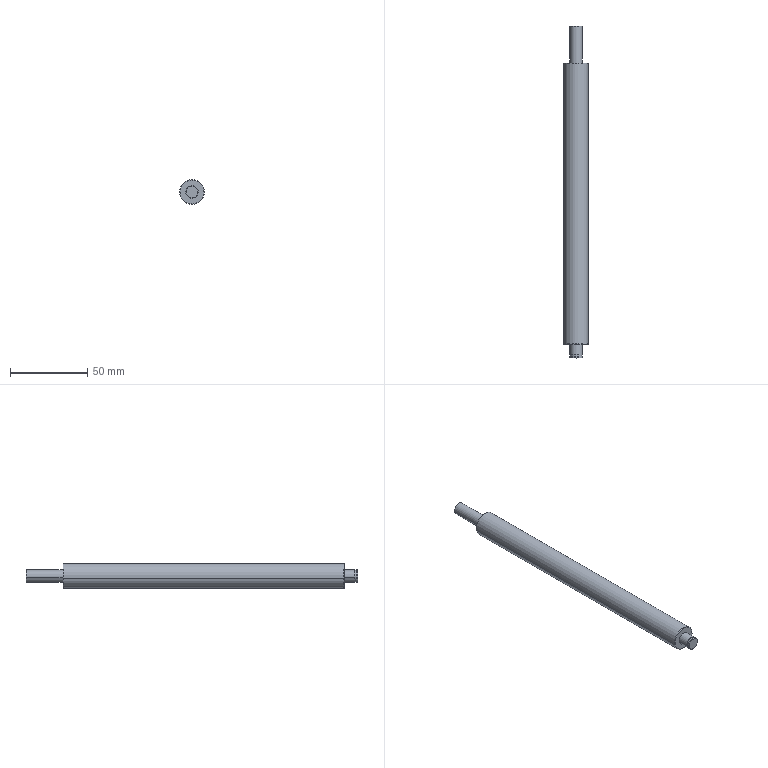Component | SolidWorks | 100-1_Copy(3)-1 | 1 solid | 24 faces | box 16 x 215 x 16 mm | volume 38242 mm3 | cylinder 10 | cone 8 | plane 6 | commonest cylinder face diameters 8 x6 7.4 x2 16 x2
STEP:
#1=COLOUR_RGB('',0.7922,0.8196,0.9333);
#2=FILL_AREA_STYLE_COLOUR('',#1);
#3=FILL_AREA_STYLE('',(#2));
#4=SURFACE_STYLE_FILL_AREA(#3);
#5=SURFACE_SIDE_STYLE('',(#4));
#6=SURFACE_STYLE_USAGE(.BOTH.,#5);
#7=PRESENTATION_STYLE_ASSIGNMENT((#6));
#8=CARTESIAN_POINT('',(19.273,49.724,-79.116));
#9=VERTEX_POINT('',#8);
#10=CARTESIAN_POINT('',(19.265,49.717,-79.117));
#11=VERTEX_POINT('',#10);
#12=CARTESIAN_POINT('',(19.273,49.724,-79.116));
#13=DIRECTION('',(-0.6974,-0.7071,-0.1169));
#14=VECTOR('',#13,39.37);
#15=LINE('',#12,#14);
#16=EDGE_CURVE('',#9,#11,#15,.T.);
#17=ORIENTED_EDGE('',*,*,#16,.F.);
#18=CARTESIAN_POINT('',(19.879,49.724,-79.014));
#19=VERTEX_POINT('',#18);
#20=CARTESIAN_POINT('',(19.576,49.724,-79.065));
#21=DIRECTION('',(-0.,1.,0.));
#22=DIRECTION('',(-0.9862,0.,-0.1654));
#23=AXIS2_PLACEMENT_3D('',#20,#21,#22);
#24=CIRCLE('',#23,0.3071);
#25=EDGE_CURVE('',#19,#9,#24,.T.);
#26=ORIENTED_EDGE('',*,*,#25,.F.);
#27=CARTESIAN_POINT('',(19.887,49.717,-79.013));
#28=VERTEX_POINT('',#27);
#29=CARTESIAN_POINT('',(19.879,49.724,-79.014));
#30=DIRECTION('',(0.6974,-0.7071,0.1169));
#31=VECTOR('',#30,39.37);
#32=LINE('',#29,#31);
#33=EDGE_CURVE('',#19,#28,#32,.T.);
#34=ORIENTED_EDGE('',*,*,#33,.T.);
#35=CARTESIAN_POINT('',(19.576,49.717,-79.065));
#36=DIRECTION('',(0.,-1.,-0.));
#37=DIRECTION('',(-0.9862,0.,-0.1654));
#38=AXIS2_PLACEMENT_3D('',#35,#36,#37);
#39=CIRCLE('',#38,0.315);
#40=EDGE_CURVE('',#11,#28,#39,.T.);
#41=ORIENTED_EDGE('',*,*,#40,.F.);
#42=EDGE_LOOP('',(#17,#26,#34,#41));
#43=FACE_OUTER_BOUND('',#42,.T.);
#44=CARTESIAN_POINT('',(19.576,49.724,-79.065));
#45=DIRECTION('',(0.,-1.,-0.));
#46=DIRECTION('',(0.9862,0.,0.1654));
#47=AXIS2_PLACEMENT_3D('',#44,#45,#46);
#48=CONICAL_SURFACE('',#47,0.3071,0.7854);
#49=ADVANCED_FACE('',(#43),#48,.T.);
#50=CARTESIAN_POINT('',(19.429,50.669,-79.09));
#51=VERTEX_POINT('',#50);
#52=CARTESIAN_POINT('',(19.421,50.661,-79.091));
#53=VERTEX_POINT('',#52);
#54=CARTESIAN_POINT('',(19.421,50.661,-79.091));
#55=DIRECTION('',(-0.6974,-0.7071,-0.1169));
#56=VECTOR('',#55,39.37);
#57=LINE('',#54,#56);
#58=EDGE_CURVE('',#51,#53,#57,.T.);
#59=ORIENTED_EDGE('',*,*,#58,.F.);
#60=CARTESIAN_POINT('',(19.724,50.669,-79.04));
#61=VERTEX_POINT('',#60);
#62=CARTESIAN_POINT('',(19.576,50.669,-79.065));
#63=DIRECTION('',(-0.,1.,0.));
#64=DIRECTION('',(-0.9862,0.,-0.1654));
#65=AXIS2_PLACEMENT_3D('',#62,#63,#64);
#66=CIRCLE('',#65,0.1496);
#67=EDGE_CURVE('',#61,#51,#66,.T.);
#68=ORIENTED_EDGE('',*,*,#67,.F.);
#69=CARTESIAN_POINT('',(19.731,50.661,-79.039));
#70=VERTEX_POINT('',#69);
#71=CARTESIAN_POINT('',(19.731,50.661,-79.039));
#72=DIRECTION('',(0.6974,-0.7071,0.1169));
#73=VECTOR('',#72,39.37);
#74=LINE('',#71,#73);
#75=EDGE_CURVE('',#61,#70,#74,.T.);
#76=ORIENTED_EDGE('',*,*,#75,.T.);
#77=CARTESIAN_POINT('',(19.576,50.661,-79.065));
#78=DIRECTION('',(0.,-1.,-0.));
#79=DIRECTION('',(-0.9862,0.,-0.1654));
#80=AXIS2_PLACEMENT_3D('',#77,#78,#79);
#81=CIRCLE('',#80,0.1575);
#82=EDGE_CURVE('',#53,#70,#81,.T.);
#83=ORIENTED_EDGE('',*,*,#82,.F.);
#84=EDGE_LOOP('',(#59,#68,#76,#83));
#85=FACE_OUTER_BOUND('',#84,.T.);
#86=CARTESIAN_POINT('',(19.576,50.661,-79.065));
#87=DIRECTION('',(0.,-1.,-0.));
#88=DIRECTION('',(0.9862,0.,0.1654));
#89=AXIS2_PLACEMENT_3D('',#86,#87,#88);
#90=CONICAL_SURFACE('',#89,0.1575,0.7854);
#91=ADVANCED_FACE('',(#85),#90,.T.);
#92=ORIENTED_EDGE('',*,*,#67,.T.);
#93=CARTESIAN_POINT('',(19.576,50.669,-79.065));
#94=DIRECTION('',(-0.,1.,0.));
#95=DIRECTION('',(-0.9862,0.,-0.1654));
#96=AXIS2_PLACEMENT_3D('',#93,#94,#95);
#97=CIRCLE('',#96,0.1496);
#98=EDGE_CURVE('',#51,#61,#97,.T.);
#99=ORIENTED_EDGE('',*,*,#98,.T.);
#100=EDGE_LOOP('',(#92,#99));
#101=FACE_OUTER_BOUND('',#100,.T.);
#102=CARTESIAN_POINT('',(19.576,50.669,-79.065));
#103=DIRECTION('',(-0.,1.,0.));
#104=DIRECTION('',(-0.9862,-0.,-0.1654));
#105=AXIS2_PLACEMENT_3D('',#102,#103,#104);
#106=PLANE('',#105);
#107=ADVANCED_FACE('',(#101),#106,.T.);
#108=CARTESIAN_POINT('',(19.421,49.724,-79.091));
#109=VERTEX_POINT('',#108);
#110=CARTESIAN_POINT('',(19.421,50.669,-79.091));
#111=DIRECTION('',(0.,-1.,-0.));
#112=VECTOR('',#111,39.37);
#113=LINE('',#110,#112);
#114=EDGE_CURVE('',#53,#109,#113,.T.);
#115=ORIENTED_EDGE('',*,*,#114,.F.);
#116=ORIENTED_EDGE('',*,*,#82,.T.);
#117=CARTESIAN_POINT('',(19.731,49.724,-79.039));
#118=VERTEX_POINT('',#117);
#119=CARTESIAN_POINT('',(19.731,50.669,-79.039));
#120=DIRECTION('',(0.,-1.,-0.));
#121=VECTOR('',#120,39.37);
#122=LINE('',#119,#121);
#123=EDGE_CURVE('',#70,#118,#122,.T.);
#124=ORIENTED_EDGE('',*,*,#123,.T.);
#125=CARTESIAN_POINT('',(19.576,49.724,-79.065));
#126=DIRECTION('',(0.,-1.,-0.));
#127=DIRECTION('',(0.9862,0.,0.1654));
#128=AXIS2_PLACEMENT_3D('',#125,#126,#127);
#129=CIRCLE('',#128,0.1575);
#130=EDGE_CURVE('',#109,#118,#129,.T.);
#131=ORIENTED_EDGE('',*,*,#130,.F.);
#132=EDGE_LOOP('',(#115,#116,#124,#131));
#133=FACE_OUTER_BOUND('',#132,.T.);
#134=CARTESIAN_POINT('',(19.576,50.669,-79.065));
#135=DIRECTION('',(0.,-1.,-0.));
#136=DIRECTION('',(0.9862,0.,0.1654));
#137=AXIS2_PLACEMENT_3D('',#134,#135,#136);
#138=CYLINDRICAL_SURFACE('',#137,0.1575);
#139=ADVANCED_FACE('',(#133),#138,.T.);
#140=CARTESIAN_POINT('',(19.576,49.724,-79.065));
#141=DIRECTION('',(0.,-1.,-0.));
#142=DIRECTION('',(0.9862,0.,0.1654));
#143=AXIS2_PLACEMENT_3D('',#140,#141,#142);
#144=CIRCLE('',#143,0.1575);
#145=EDGE_CURVE('',#118,#109,#144,.T.);
#146=ORIENTED_EDGE('',*,*,#145,.T.);
#147=ORIENTED_EDGE('',*,*,#130,.T.);
#148=EDGE_LOOP('',(#146,#147));
#149=FACE_BOUND('',#148,.T.);
#150=ORIENTED_EDGE('',*,*,#25,.T.);
#151=CARTESIAN_POINT('',(19.576,49.724,-79.065));
#152=DIRECTION('',(-0.,1.,0.));
#153=DIRECTION('',(-0.9862,0.,-0.1654));
#154=AXIS2_PLACEMENT_3D('',#151,#152,#153);
#155=CIRCLE('',#154,0.3071);
#156=EDGE_CURVE('',#9,#19,#155,.T.);
#157=ORIENTED_EDGE('',*,*,#156,.T.);
#158=EDGE_LOOP('',(#150,#157));
#159=FACE_OUTER_BOUND('',#158,.T.);
#160=CARTESIAN_POINT('',(18.655,49.724,-79.219));
#161=DIRECTION('',(-0.,1.,0.));
#162=DIRECTION('',(-0.9862,-0.,-0.1654));
#163=AXIS2_PLACEMENT_3D('',#160,#161,#162);
#164=PLANE('',#163);
#165=ADVANCED_FACE('',(#149,#159),#164,.T.);
#166=CARTESIAN_POINT('',(19.421,42.244,-79.091));
#167=VERTEX_POINT('',#166);
#168=CARTESIAN_POINT('',(19.421,42.213,-79.091));
#169=VERTEX_POINT('',#168);
#170=CARTESIAN_POINT('',(19.421,42.205,-79.091));
#171=DIRECTION('',(0.,-1.,-0.));
#172=VECTOR('',#171,39.37);
#173=LINE('',#170,#172);
#174=EDGE_CURVE('',#167,#169,#173,.T.);
#175=ORIENTED_EDGE('',*,*,#174,.F.);
#176=CARTESIAN_POINT('',(19.731,42.244,-79.039));
#177=VERTEX_POINT('',#176);
#178=CARTESIAN_POINT('',(19.576,42.244,-79.065));
#179=DIRECTION('',(-0.,1.,0.));
#180=DIRECTION('',(0.9862,0.,0.1654));
#181=AXIS2_PLACEMENT_3D('',#178,#179,#180);
#182=CIRCLE('',#181,0.1575);
#183=EDGE_CURVE('',#177,#167,#182,.T.);
#184=ORIENTED_EDGE('',*,*,#183,.F.);
#185=CARTESIAN_POINT('',(19.731,42.213,-79.039));
#186=VERTEX_POINT('',#185);
#187=CARTESIAN_POINT('',(19.731,42.205,-79.039));
#188=DIRECTION('',(0.,-1.,-0.));
#189=VECTOR('',#188,39.37);
#190=LINE('',#187,#189);
#191=EDGE_CURVE('',#177,#186,#190,.T.);
#192=ORIENTED_EDGE('',*,*,#191,.T.);
#193=CARTESIAN_POINT('',(19.576,42.213,-79.065));
#194=DIRECTION('',(-0.,1.,0.));
#195=DIRECTION('',(-0.9862,0.,-0.1654));
#196=AXIS2_PLACEMENT_3D('',#193,#194,#195);
#197=CIRCLE('',#196,0.1575);
#198=EDGE_CURVE('',#186,#169,#197,.T.);
#199=ORIENTED_EDGE('',*,*,#198,.T.);
#200=EDGE_LOOP('',(#175,#184,#192,#199));
#201=FACE_OUTER_BOUND('',#200,.T.);
#202=CARTESIAN_POINT('',(19.576,42.205,-79.065));
#203=DIRECTION('',(0.,-1.,-0.));
#204=DIRECTION('',(0.9862,0.,0.1654));
#205=AXIS2_PLACEMENT_3D('',#202,#203,#204);
#206=CYLINDRICAL_SURFACE('',#205,0.1575);
#207=ADVANCED_FACE('',(#201),#206,.T.);
#208=CARTESIAN_POINT('',(19.724,42.205,-79.04));
#209=VERTEX_POINT('',#208);
#210=CARTESIAN_POINT('',(19.731,42.213,-79.039));
#211=DIRECTION('',(0.6974,0.7071,0.1169));
#212=VECTOR('',#211,39.37);
#213=LINE('',#210,#212);
#214=EDGE_CURVE('',#209,#186,#213,.T.);
#215=ORIENTED_EDGE('',*,*,#214,.F.);
#216=CARTESIAN_POINT('',(19.429,42.205,-79.09));
#217=VERTEX_POINT('',#216);
#218=CARTESIAN_POINT('',(19.576,42.205,-79.065));
#219=DIRECTION('',(0.,-1.,-0.));
#220=DIRECTION('',(-0.9862,0.,-0.1654));
#221=AXIS2_PLACEMENT_3D('',#218,#219,#220);
#222=CIRCLE('',#221,0.1496);
#223=EDGE_CURVE('',#217,#209,#222,.T.);
#224=ORIENTED_EDGE('',*,*,#223,.F.);
#225=CARTESIAN_POINT('',(19.421,42.213,-79.091));
#226=DIRECTION('',(-0.6974,0.7071,-0.1169));
#227=VECTOR('',#226,39.37);
#228=LINE('',#225,#227);
#229=EDGE_CURVE('',#217,#169,#228,.T.);
#230=ORIENTED_EDGE('',*,*,#229,.T.);
#231=ORIENTED_EDGE('',*,*,#198,.F.);
#232=EDGE_LOOP('',(#215,#224,#230,#231));
#233=FACE_OUTER_BOUND('',#232,.T.);
#234=CARTESIAN_POINT('',(19.576,42.213,-79.065));
#235=DIRECTION('',(-0.,1.,0.));
#236=DIRECTION('',(-0.9862,0.,-0.1654));
#237=AXIS2_PLACEMENT_3D('',#234,#235,#236);
#238=CONICAL_SURFACE('',#237,0.1575,0.7854);
#239=ADVANCED_FACE('',(#233),#238,.T.);
#240=ORIENTED_EDGE('',*,*,#223,.T.);
#241=CARTESIAN_POINT('',(19.576,42.205,-79.065));
#242=DIRECTION('',(0.,-1.,-0.));
#243=DIRECTION('',(-0.9862,0.,-0.1654));
#244=AXIS2_PLACEMENT_3D('',#241,#242,#243);
#245=CIRCLE('',#244,0.1496);
#246=EDGE_CURVE('',#209,#217,#245,.T.);
#247=ORIENTED_EDGE('',*,*,#246,.T.);
#248=EDGE_LOOP('',(#240,#247));
#249=FACE_OUTER_BOUND('',#248,.T.);
#250=CARTESIAN_POINT('',(19.576,42.205,-79.065));
#251=DIRECTION('',(-0.,1.,0.));
#252=DIRECTION('',(-0.9862,-0.,-0.1654));
#253=AXIS2_PLACEMENT_3D('',#250,#251,#252);
#254=PLANE('',#253);
#255=ADVANCED_FACE('',(#249),#254,.F.);
#256=CARTESIAN_POINT('',(19.432,42.283,-79.089));
#257=VERTEX_POINT('',#256);
#258=CARTESIAN_POINT('',(19.72,42.283,-79.041));
#259=VERTEX_POINT('',#258);
#260=CARTESIAN_POINT('',(19.576,42.283,-79.065));
#261=DIRECTION('',(-0.,1.,0.));
#262=DIRECTION('',(-0.9862,0.,-0.1654));
#263=AXIS2_PLACEMENT_3D('',#260,#261,#262);
#264=CIRCLE('',#263,0.1457);
#265=EDGE_CURVE('',#257,#259,#264,.T.);
#266=ORIENTED_EDGE('',*,*,#265,.T.);
#267=CARTESIAN_POINT('',(19.576,42.283,-79.065));
#268=DIRECTION('',(-0.,1.,0.));
#269=DIRECTION('',(-0.9862,0.,-0.1654));
#270=AXIS2_PLACEMENT_3D('',#267,#268,#269);
#271=CIRCLE('',#270,0.1457);
#272=EDGE_CURVE('',#259,#257,#271,.T.);
#273=ORIENTED_EDGE('',*,*,#272,.T.);
#274=EDGE_LOOP('',(#266,#273));
#275=FACE_BOUND('',#274,.T.);
#276=CARTESIAN_POINT('',(19.731,42.283,-79.039));
#277=VERTEX_POINT('',#276);
#278=CARTESIAN_POINT('',(19.421,42.283,-79.091));
#279=VERTEX_POINT('',#278);
#280=CARTESIAN_POINT('',(19.576,42.283,-79.065));
#281=DIRECTION('',(0.,-1.,-0.));
#282=DIRECTION('',(-0.9862,0.,-0.1654));
#283=AXIS2_PLACEMENT_3D('',#280,#281,#282);
#284=CIRCLE('',#283,0.1575);
#285=EDGE_CURVE('',#277,#279,#284,.T.);
#286=ORIENTED_EDGE('',*,*,#285,.T.);
#287=CARTESIAN_POINT('',(19.576,42.283,-79.065));
#288=DIRECTION('',(0.,-1.,-0.));
#289=DIRECTION('',(-0.9862,0.,-0.1654));
#290=AXIS2_PLACEMENT_3D('',#287,#288,#289);
#291=CIRCLE('',#290,0.1575);
#292=EDGE_CURVE('',#279,#277,#291,.T.);
#293=ORIENTED_EDGE('',*,*,#292,.T.);
#294=EDGE_LOOP('',(#286,#293));
#295=FACE_OUTER_BOUND('',#294,.T.);
#296=CARTESIAN_POINT('',(19.432,42.283,-79.089));
#297=DIRECTION('',(-0.,1.,0.));
#298=DIRECTION('',(-0.9862,-0.,-0.1654));
#299=AXIS2_PLACEMENT_3D('',#296,#297,#298);
#300=PLANE('',#299);
#301=ADVANCED_FACE('',(#275,#295),#300,.F.);
#302=CARTESIAN_POINT('',(19.72,42.244,-79.041));
#303=VERTEX_POINT('',#302);
#304=CARTESIAN_POINT('',(19.72,42.205,-79.041));
#305=DIRECTION('',(-0.,1.,0.));
#306=VECTOR('',#305,39.37);
#307=LINE('',#304,#306);
#308=EDGE_CURVE('',#303,#259,#307,.T.);
#309=ORIENTED_EDGE('',*,*,#308,.F.);
#310=CARTESIAN_POINT('',(19.432,42.244,-79.089));
#311=VERTEX_POINT('',#310);
#312=CARTESIAN_POINT('',(19.576,42.244,-79.065));
#313=DIRECTION('',(-0.,1.,0.));
#314=DIRECTION('',(-0.9862,0.,-0.1654));
#315=AXIS2_PLACEMENT_3D('',#312,#313,#314);
#316=CIRCLE('',#315,0.1457);
#317=EDGE_CURVE('',#303,#311,#316,.T.);
#318=ORIENTED_EDGE('',*,*,#317,.T.);
#319=CARTESIAN_POINT('',(19.432,42.205,-79.089));
#320=DIRECTION('',(-0.,1.,0.));
#321=VECTOR('',#320,39.37);
#322=LINE('',#319,#321);
#323=EDGE_CURVE('',#311,#257,#322,.T.);
#324=ORIENTED_EDGE('',*,*,#323,.T.);
#325=ORIENTED_EDGE('',*,*,#272,.F.);
#326=EDGE_LOOP('',(#309,#318,#324,#325));
#327=FACE_OUTER_BOUND('',#326,.T.);
#328=CARTESIAN_POINT('',(19.576,42.205,-79.065));
#329=DIRECTION('',(-0.,1.,0.));
#330=DIRECTION('',(-0.9862,0.,-0.1654));
#331=AXIS2_PLACEMENT_3D('',#328,#329,#330);
#332=CYLINDRICAL_SURFACE('',#331,0.1457);
#333=ADVANCED_FACE('',(#327),#332,.T.);
#334=CARTESIAN_POINT('',(19.576,42.244,-79.065));
#335=DIRECTION('',(-0.,1.,0.));
#336=DIRECTION('',(-0.9862,0.,-0.1654));
#337=AXIS2_PLACEMENT_3D('',#334,#335,#336);
#338=CIRCLE('',#337,0.1457);
#339=EDGE_CURVE('',#311,#303,#338,.T.);
#340=ORIENTED_EDGE('',*,*,#339,.F.);
#341=ORIENTED_EDGE('',*,*,#317,.F.);
#342=EDGE_LOOP('',(#340,#341));
#343=FACE_BOUND('',#342,.T.);
#344=ORIENTED_EDGE('',*,*,#183,.T.);
#345=CARTESIAN_POINT('',(19.576,42.244,-79.065));
#346=DIRECTION('',(-0.,1.,0.));
#347=DIRECTION('',(0.9862,0.,0.1654));
#348=AXIS2_PLACEMENT_3D('',#345,#346,#347);
#349=CIRCLE('',#348,0.1575);
#350=EDGE_CURVE('',#167,#177,#349,.T.);
#351=ORIENTED_EDGE('',*,*,#350,.T.);
#352=EDGE_LOOP('',(#344,#351));
#353=FACE_OUTER_BOUND('',#352,.T.);
#354=CARTESIAN_POINT('',(19.432,42.244,-79.089));
#355=DIRECTION('',(0.,-1.,-0.));
#356=DIRECTION('',(0.1654,0.,-0.9862));
#357=AXIS2_PLACEMENT_3D('',#354,#355,#356);
#358=PLANE('',#357);
#359=ADVANCED_FACE('',(#343,#353),#358,.F.);
#360=CARTESIAN_POINT('',(19.879,42.559,-79.014));
#361=VERTEX_POINT('',#360);
#362=CARTESIAN_POINT('',(19.887,42.567,-79.013));
#363=VERTEX_POINT('',#362);
#364=CARTESIAN_POINT('',(19.879,42.559,-79.014));
#365=DIRECTION('',(0.6974,0.7071,0.1169));
#366=VECTOR('',#365,39.37);
#367=LINE('',#364,#366);
#368=EDGE_CURVE('',#361,#363,#367,.T.);
#369=ORIENTED_EDGE('',*,*,#368,.F.);
#370=CARTESIAN_POINT('',(19.273,42.559,-79.116));
#371=VERTEX_POINT('',#370);
#372=CARTESIAN_POINT('',(19.576,42.559,-79.065));
#373=DIRECTION('',(0.,-1.,-0.));
#374=DIRECTION('',(0.9862,0.,0.1654));
#375=AXIS2_PLACEMENT_3D('',#372,#373,#374);
#376=CIRCLE('',#375,0.3071);
#377=EDGE_CURVE('',#371,#361,#376,.T.);
#378=ORIENTED_EDGE('',*,*,#377,.F.);
#379=CARTESIAN_POINT('',(19.265,42.567,-79.117));
#380=VERTEX_POINT('',#379);
#381=CARTESIAN_POINT('',(19.273,42.559,-79.116));
#382=DIRECTION('',(-0.6974,0.7071,-0.1169));
#383=VECTOR('',#382,39.37);
#384=LINE('',#381,#383);
#385=EDGE_CURVE('',#371,#380,#384,.T.);
#386=ORIENTED_EDGE('',*,*,#385,.T.);
#387=CARTESIAN_POINT('',(19.576,42.567,-79.065));
#388=DIRECTION('',(-0.,1.,0.));
#389=DIRECTION('',(0.9862,0.,0.1654));
#390=AXIS2_PLACEMENT_3D('',#387,#388,#389);
#391=CIRCLE('',#390,0.315);
#392=EDGE_CURVE('',#363,#380,#391,.T.);
#393=ORIENTED_EDGE('',*,*,#392,.F.);
#394=EDGE_LOOP('',(#369,#378,#386,#393));
#395=FACE_OUTER_BOUND('',#394,.T.);
#396=CARTESIAN_POINT('',(19.576,42.559,-79.065));
#397=DIRECTION('',(-0.,1.,0.));
#398=DIRECTION('',(-0.9862,0.,-0.1654));
#399=AXIS2_PLACEMENT_3D('',#396,#397,#398);
#400=CONICAL_SURFACE('',#399,0.3071,0.7854);
#401=ADVANCED_FACE('',(#395),#400,.T.);
#402=CARTESIAN_POINT('',(19.421,42.559,-79.091));
#403=VERTEX_POINT('',#402);
#404=CARTESIAN_POINT('',(19.421,42.205,-79.091));
#405=DIRECTION('',(0.,-1.,-0.));
#406=VECTOR('',#405,39.37);
#407=LINE('',#404,#406);
#408=EDGE_CURVE('',#403,#279,#407,.T.);
#409=ORIENTED_EDGE('',*,*,#408,.F.);
#410=CARTESIAN_POINT('',(19.731,42.559,-79.039));
#411=VERTEX_POINT('',#410);
#412=CARTESIAN_POINT('',(19.576,42.559,-79.065));
#413=DIRECTION('',(0.,-1.,-0.));
#414=DIRECTION('',(0.9862,0.,0.1654));
#415=AXIS2_PLACEMENT_3D('',#412,#413,#414);
#416=CIRCLE('',#415,0.1575);
#417=EDGE_CURVE('',#403,#411,#416,.T.);
#418=ORIENTED_EDGE('',*,*,#417,.T.);
#419=CARTESIAN_POINT('',(19.731,42.205,-79.039));
#420=DIRECTION('',(0.,-1.,-0.));
#421=VECTOR('',#420,39.37);
#422=LINE('',#419,#421);
#423=EDGE_CURVE('',#411,#277,#422,.T.);
#424=ORIENTED_EDGE('',*,*,#423,.T.);
#425=ORIENTED_EDGE('',*,*,#292,.F.);
#426=EDGE_LOOP('',(#409,#418,#424,#425));
#427=FACE_OUTER_BOUND('',#426,.T.);
#428=CARTESIAN_POINT('',(19.576,42.205,-79.065));
#429=DIRECTION('',(0.,-1.,-0.));
#430=DIRECTION('',(0.9862,0.,0.1654));
#431=AXIS2_PLACEMENT_3D('',#428,#429,#430);
#432=CYLINDRICAL_SURFACE('',#431,0.1575);
#433=ADVANCED_FACE('',(#427),#432,.T.);
#434=CARTESIAN_POINT('',(19.576,42.559,-79.065));
#435=DIRECTION('',(0.,-1.,-0.));
#436=DIRECTION('',(0.9862,0.,0.1654));
#437=AXIS2_PLACEMENT_3D('',#434,#435,#436);
#438=CIRCLE('',#437,0.1575);
#439=EDGE_CURVE('',#411,#403,#438,.T.);
#440=ORIENTED_EDGE('',*,*,#439,.F.);
#441=ORIENTED_EDGE('',*,*,#417,.F.);
#442=EDGE_LOOP('',(#440,#441));
#443=FACE_BOUND('',#442,.T.);
#444=ORIENTED_EDGE('',*,*,#377,.T.);
#445=CARTESIAN_POINT('',(19.576,42.559,-79.065));
#446=DIRECTION('',(0.,-1.,-0.));
#447=DIRECTION('',(0.9862,0.,0.1654));
#448=AXIS2_PLACEMENT_3D('',#445,#446,#447);
#449=CIRCLE('',#448,0.3071);
#450=EDGE_CURVE('',#361,#371,#449,.T.);
#451=ORIENTED_EDGE('',*,*,#450,.T.);
#452=EDGE_LOOP('',(#444,#451));
#453=FACE_OUTER_BOUND('',#452,.T.);
#454=CARTESIAN_POINT('',(19.077,42.559,-79.149));
#455=DIRECTION('',(0.,-1.,-0.));
#456=DIRECTION('',(0.1654,0.,-0.9862));
#457=AXIS2_PLACEMENT_3D('',#454,#455,#456);
#458=PLANE('',#457);
#459=ADVANCED_FACE('',(#443,#453),#458,.T.);
#460=CARTESIAN_POINT('',(19.265,50.669,-79.117));
#461=DIRECTION('',(0.,-1.,-0.));
#462=VECTOR('',#461,39.37);
#463=LINE('',#460,#462);
#464=EDGE_CURVE('',#11,#380,#463,.T.);
#465=ORIENTED_EDGE('',*,*,#464,.F.);
#466=ORIENTED_EDGE('',*,*,#40,.T.);
#467=CARTESIAN_POINT('',(19.887,50.669,-79.013));
#468=DIRECTION('',(0.,-1.,-0.));
#469=VECTOR('',#468,39.37);
#470=LINE('',#467,#469);
#471=EDGE_CURVE('',#28,#363,#470,.T.);
#472=ORIENTED_EDGE('',*,*,#471,.T.);
#473=ORIENTED_EDGE('',*,*,#392,.T.);
#474=EDGE_LOOP('',(#465,#466,#472,#473));
#475=FACE_OUTER_BOUND('',#474,.T.);
#476=CARTESIAN_POINT('',(19.576,50.669,-79.065));
#477=DIRECTION('',(0.,-1.,-0.));
#478=DIRECTION('',(0.9862,0.,0.1654));
#479=AXIS2_PLACEMENT_3D('',#476,#477,#478);
#480=CYLINDRICAL_SURFACE('',#479,0.315);
#481=ADVANCED_FACE('',(#475),#480,.T.);
#482=CARTESIAN_POINT('',(19.576,49.717,-79.065));
#483=DIRECTION('',(0.,-1.,-0.));
#484=DIRECTION('',(-0.9862,0.,-0.1654));
#485=AXIS2_PLACEMENT_3D('',#482,#483,#484);
#486=CIRCLE('',#485,0.315);
#487=EDGE_CURVE('',#28,#11,#486,.T.);
#488=ORIENTED_EDGE('',*,*,#487,.T.);
#489=ORIENTED_EDGE('',*,*,#464,.T.);
#490=CARTESIAN_POINT('',(19.576,42.567,-79.065));
#491=DIRECTION('',(-0.,1.,0.));
#492=DIRECTION('',(0.9862,0.,0.1654));
#493=AXIS2_PLACEMENT_3D('',#490,#491,#492);
#494=CIRCLE('',#493,0.315);
#495=EDGE_CURVE('',#380,#363,#494,.T.);
#496=ORIENTED_EDGE('',*,*,#495,.T.);
#497=ORIENTED_EDGE('',*,*,#471,.F.);
#498=EDGE_LOOP('',(#488,#489,#496,#497));
#499=FACE_OUTER_BOUND('',#498,.T.);
#500=CARTESIAN_POINT('',(19.576,50.669,-79.065));
#501=DIRECTION('',(0.,-1.,-0.));
#502=DIRECTION('',(0.9862,0.,0.1654));
#503=AXIS2_PLACEMENT_3D('',#500,#501,#502);
#504=CYLINDRICAL_SURFACE('',#503,0.315);
#505=ADVANCED_FACE('',(#499),#504,.T.);
#506=ORIENTED_EDGE('',*,*,#439,.T.);
#507=ORIENTED_EDGE('',*,*,#408,.T.);
#508=ORIENTED_EDGE('',*,*,#285,.F.);
#509=ORIENTED_EDGE('',*,*,#423,.F.);
#510=EDGE_LOOP('',(#506,#507,#508,#509));
#511=FACE_OUTER_BOUND('',#510,.T.);
#512=CARTESIAN_POINT('',(19.576,42.205,-79.065));
#513=DIRECTION('',(0.,-1.,-0.));
#514=DIRECTION('',(0.9862,0.,0.1654));
#515=AXIS2_PLACEMENT_3D('',#512,#513,#514);
#516=CYLINDRICAL_SURFACE('',#515,0.1575);
#517=ADVANCED_FACE('',(#511),#516,.T.);
#518=ORIENTED_EDGE('',*,*,#450,.F.);
#519=ORIENTED_EDGE('',*,*,#368,.T.);
#520=ORIENTED_EDGE('',*,*,#495,.F.);
#521=ORIENTED_EDGE('',*,*,#385,.F.);
#522=EDGE_LOOP('',(#518,#519,#520,#521));
#523=FACE_OUTER_BOUND('',#522,.T.);
#524=CARTESIAN_POINT('',(19.576,42.559,-79.065));
#525=DIRECTION('',(-0.,1.,0.));
#526=DIRECTION('',(-0.9862,0.,-0.1654));
#527=AXIS2_PLACEMENT_3D('',#524,#525,#526);
#528=CONICAL_SURFACE('',#527,0.3071,0.7854);
#529=ADVANCED_FACE('',(#523),#528,.T.);
#530=ORIENTED_EDGE('',*,*,#339,.T.);
#531=ORIENTED_EDGE('',*,*,#308,.T.);
#532=ORIENTED_EDGE('',*,*,#265,.F.);
#533=ORIENTED_EDGE('',*,*,#323,.F.);
#534=EDGE_LOOP('',(#530,#531,#532,#533));
#535=FACE_OUTER_BOUND('',#534,.T.);
#536=CARTESIAN_POINT('',(19.576,42.205,-79.065));
#537=DIRECTION('',(-0.,1.,0.));
#538=DIRECTION('',(-0.9862,0.,-0.1654));
#539=AXIS2_PLACEMENT_3D('',#536,#537,#538);
#540=CYLINDRICAL_SURFACE('',#539,0.1457);
#541=ADVANCED_FACE('',(#535),#540,.T.);
#542=ORIENTED_EDGE('',*,*,#246,.F.);
#543=ORIENTED_EDGE('',*,*,#214,.T.);
#544=CARTESIAN_POINT('',(19.576,42.213,-79.065));
#545=DIRECTION('',(-0.,1.,0.));
#546=DIRECTION('',(-0.9862,0.,-0.1654));
#547=AXIS2_PLACEMENT_3D('',#544,#545,#546);
#548=CIRCLE('',#547,0.1575);
#549=EDGE_CURVE('',#169,#186,#548,.T.);
#550=ORIENTED_EDGE('',*,*,#549,.F.);
#551=ORIENTED_EDGE('',*,*,#229,.F.);
#552=EDGE_LOOP('',(#542,#543,#550,#551));
#553=FACE_OUTER_BOUND('',#552,.T.);
#554=CARTESIAN_POINT('',(19.576,42.213,-79.065));
#555=DIRECTION('',(-0.,1.,0.));
#556=DIRECTION('',(-0.9862,0.,-0.1654));
#557=AXIS2_PLACEMENT_3D('',#554,#555,#556);
#558=CONICAL_SURFACE('',#557,0.1575,0.7854);
#559=ADVANCED_FACE('',(#553),#558,.T.);
#560=ORIENTED_EDGE('',*,*,#350,.F.);
#561=ORIENTED_EDGE('',*,*,#174,.T.);
#562=ORIENTED_EDGE('',*,*,#549,.T.);
#563=ORIENTED_EDGE('',*,*,#191,.F.);
#564=EDGE_LOOP('',(#560,#561,#562,#563));
#565=FACE_OUTER_BOUND('',#564,.T.);
#566=CARTESIAN_POINT('',(19.576,42.205,-79.065));
#567=DIRECTION('',(0.,-1.,-0.));
#568=DIRECTION('',(0.9862,0.,0.1654));
#569=AXIS2_PLACEMENT_3D('',#566,#567,#568);
#570=CYLINDRICAL_SURFACE('',#569,0.1575);
#571=ADVANCED_FACE('',(#565),#570,.T.);
#572=CARTESIAN_POINT('',(19.576,50.661,-79.065));
#573=DIRECTION('',(0.,-1.,-0.));
#574=DIRECTION('',(-0.9862,0.,-0.1654));
#575=AXIS2_PLACEMENT_3D('',#572,#573,#574);
#576=CIRCLE('',#575,0.1575);
#577=EDGE_CURVE('',#70,#53,#576,.T.);
#578=ORIENTED_EDGE('',*,*,#577,.T.);
#579=ORIENTED_EDGE('',*,*,#114,.T.);
#580=ORIENTED_EDGE('',*,*,#145,.F.);
#581=ORIENTED_EDGE('',*,*,#123,.F.);
#582=EDGE_LOOP('',(#578,#579,#580,#581));
#583=FACE_OUTER_BOUND('',#582,.T.);
#584=CARTESIAN_POINT('',(19.576,50.669,-79.065));
#585=DIRECTION('',(0.,-1.,-0.));
#586=DIRECTION('',(0.9862,0.,0.1654));
#587=AXIS2_PLACEMENT_3D('',#584,#585,#586);
#588=CYLINDRICAL_SURFACE('',#587,0.1575);
#589=ADVANCED_FACE('',(#583),#588,.T.);
#590=ORIENTED_EDGE('',*,*,#98,.F.);
#591=ORIENTED_EDGE('',*,*,#58,.T.);
#592=ORIENTED_EDGE('',*,*,#577,.F.);
#593=ORIENTED_EDGE('',*,*,#75,.F.);
#594=EDGE_LOOP('',(#590,#591,#592,#593));
#595=FACE_OUTER_BOUND('',#594,.T.);
#596=CARTESIAN_POINT('',(19.576,50.661,-79.065));
#597=DIRECTION('',(0.,-1.,-0.));
#598=DIRECTION('',(0.9862,0.,0.1654));
#599=AXIS2_PLACEMENT_3D('',#596,#597,#598);
#600=CONICAL_SURFACE('',#599,0.1575,0.7854);
#601=ADVANCED_FACE('',(#595),#600,.T.);
#602=ORIENTED_EDGE('',*,*,#156,.F.);
#603=ORIENTED_EDGE('',*,*,#16,.T.);
#604=ORIENTED_EDGE('',*,*,#487,.F.);
#605=ORIENTED_EDGE('',*,*,#33,.F.);
#606=EDGE_LOOP('',(#602,#603,#604,#605));
#607=FACE_OUTER_BOUND('',#606,.T.);
#608=CARTESIAN_POINT('',(19.576,49.724,-79.065));
#609=DIRECTION('',(0.,-1.,-0.));
#610=DIRECTION('',(0.9862,0.,0.1654));
#611=AXIS2_PLACEMENT_3D('',#608,#609,#610);
#612=CONICAL_SURFACE('',#611,0.3071,0.7854);
#613=ADVANCED_FACE('',(#607),#612,.T.);
#614=CLOSED_SHELL('',(#49,#91,#107,#139,#165,#207,#239,#255,#301,#333,#359,#401,#433,#459,#481,#505,#517,#529,#541,#559,#571,#589,#601,#613));
#615=MANIFOLD_SOLID_BREP('',#614);
#616=STYLED_ITEM('',(#7),#615);
#617=PRESENTATION_LAYER_ASSIGNMENT('','',(#616));
#618=CARTESIAN_POINT('',(0.,0.,0.));
#619=DIRECTION('',(0.,0.,1.));
#620=DIRECTION('',(1.,0.,0.));
#621=AXIS2_PLACEMENT_3D('',#618,#619,#620);
#622=(LENGTH_UNIT()NAMED_UNIT(*)SI_UNIT($,.METRE.));
#623=LENGTH_MEASURE_WITH_UNIT(LENGTH_MEASURE(0.0254),#622);
#624=DIMENSIONAL_EXPONENTS(1.,0.,0.,0.,0.,0.,0.);
#625=(CONVERSION_BASED_UNIT('',#623)LENGTH_UNIT()NAMED_UNIT(#624));
#626=UNCERTAINTY_MEASURE_WITH_UNIT(LENGTH_MEASURE(0.00001),#625,'','');
#627=(NAMED_UNIT(*)PLANE_ANGLE_UNIT()SI_UNIT($,.RADIAN.));
#628=(NAMED_UNIT(*)SI_UNIT($,.STERADIAN.)SOLID_ANGLE_UNIT());
#629=(GEOMETRIC_REPRESENTATION_CONTEXT(3)GLOBAL_UNCERTAINTY_ASSIGNED_CONTEXT((#626))GLOBAL_UNIT_ASSIGNED_CONTEXT((#625,#627,#628))REPRESENTATION_CONTEXT('',''));
#630=ADVANCED_BREP_SHAPE_REPRESENTATION('',(#615,#621),#629);
#631=(LENGTH_UNIT()NAMED_UNIT(*)SI_UNIT($,.METRE.));
#632=LENGTH_MEASURE_WITH_UNIT(LENGTH_MEASURE(0.0254),#631);
#633=DIMENSIONAL_EXPONENTS(1.,0.,0.,0.,0.,0.,0.);
#634=(CONVERSION_BASED_UNIT('',#632)LENGTH_UNIT()NAMED_UNIT(#633));
#635=UNCERTAINTY_MEASURE_WITH_UNIT(LENGTH_MEASURE(0.00001),#634,'','');
#636=(NAMED_UNIT(*)PLANE_ANGLE_UNIT()SI_UNIT($,.RADIAN.));
#637=(NAMED_UNIT(*)SI_UNIT($,.STERADIAN.)SOLID_ANGLE_UNIT());
#638=(GEOMETRIC_REPRESENTATION_CONTEXT(3)GLOBAL_UNCERTAINTY_ASSIGNED_CONTEXT((#635))GLOBAL_UNIT_ASSIGNED_CONTEXT((#634,#636,#637))REPRESENTATION_CONTEXT('',''));
#639=MECHANICAL_DESIGN_GEOMETRIC_PRESENTATION_REPRESENTATION('',(#616),#638);